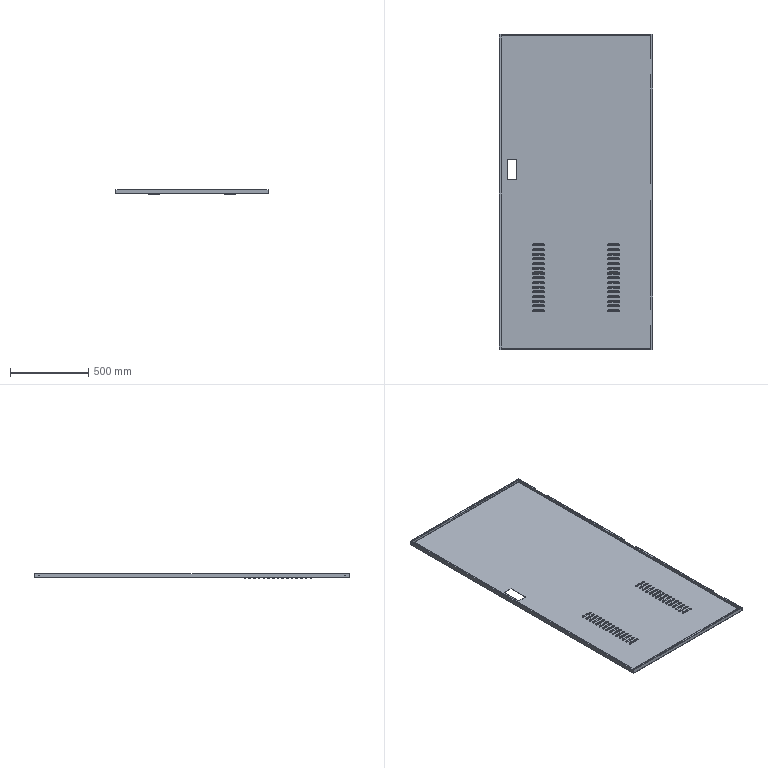Component | SolidWorks | FrontDoorPanel1-2 | 1 solid | 866 faces | volume 3264002 mm3 | cylinder 386 | plane 240 | torus 240 | commonest cylinder face diameters 8 x180 5 x90 11 x90 3.4 x13 0.4 x13